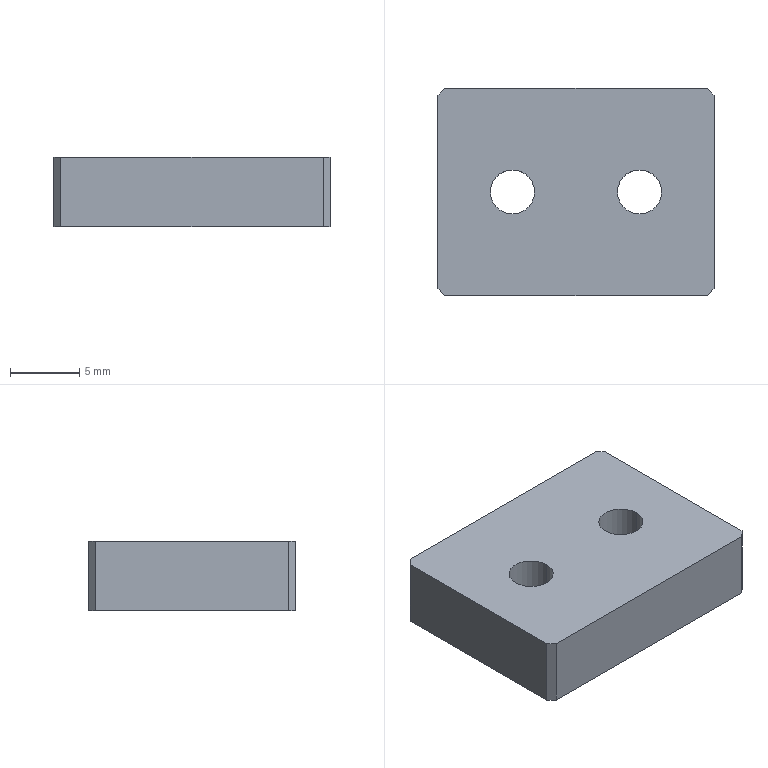CAM job | Mastercam | mm | 4 operations | part box 20 x 15 x 5
1. Helix Bore | 17 - 2 平铣刀
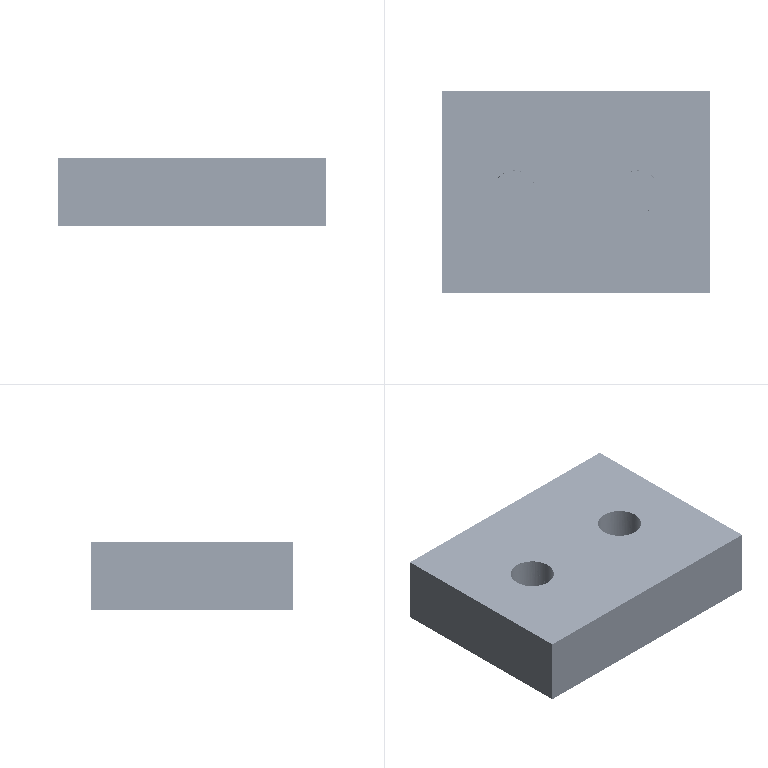2. Contour (Ramp) | 6 - 6 平底刀
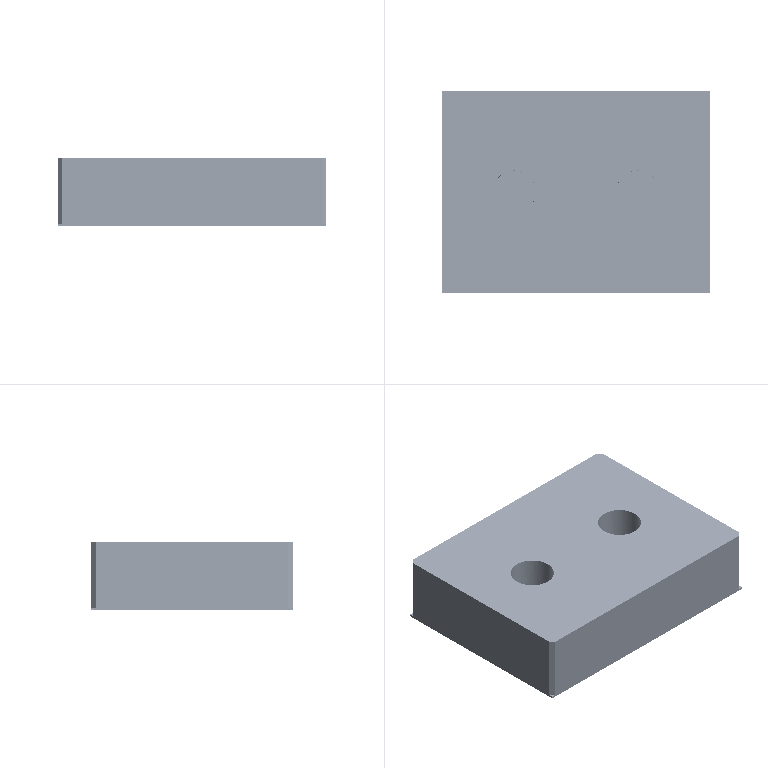3. Contour (2D) | 7 - 4 平底刀
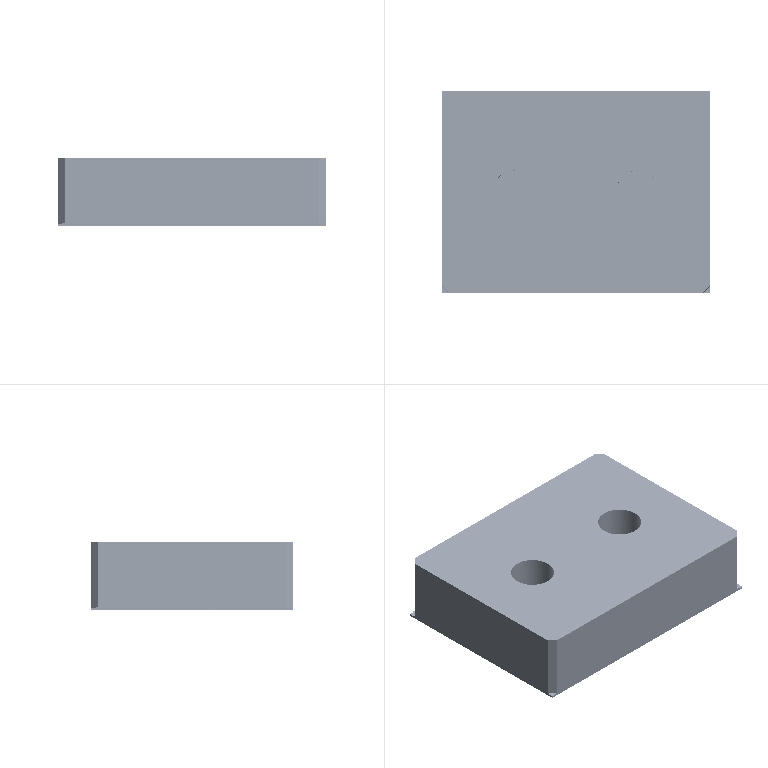4. Model Chamfer | 2 - 6定位倒角